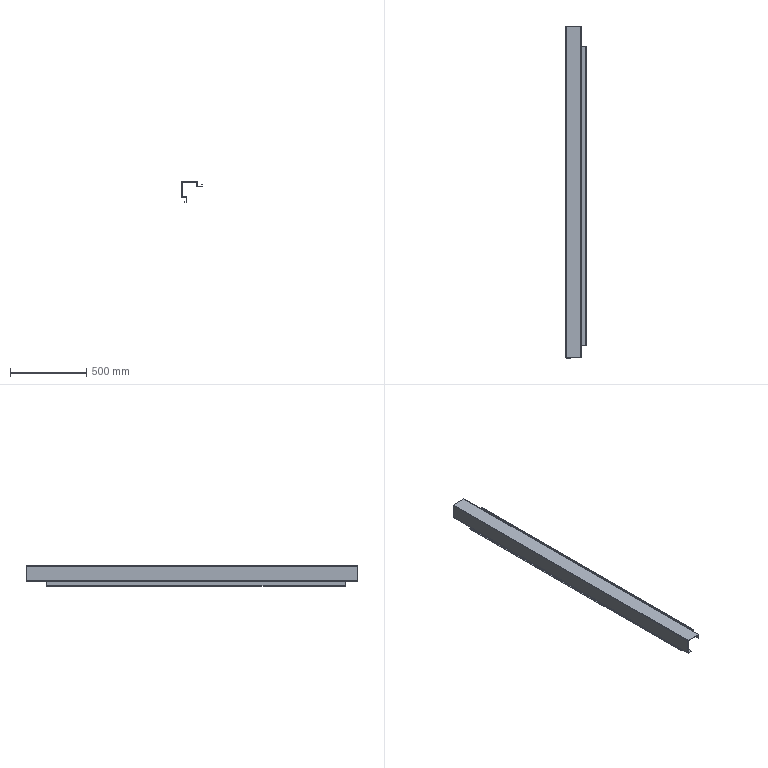Component | SolidWorks | Column-1 | 1 solid | 99 faces | volume 1068620 mm3 | plane 56 | cylinder 43 | commonest cylinder face diameters 11 x21 9 x8 3.4 x7 0.4 x7